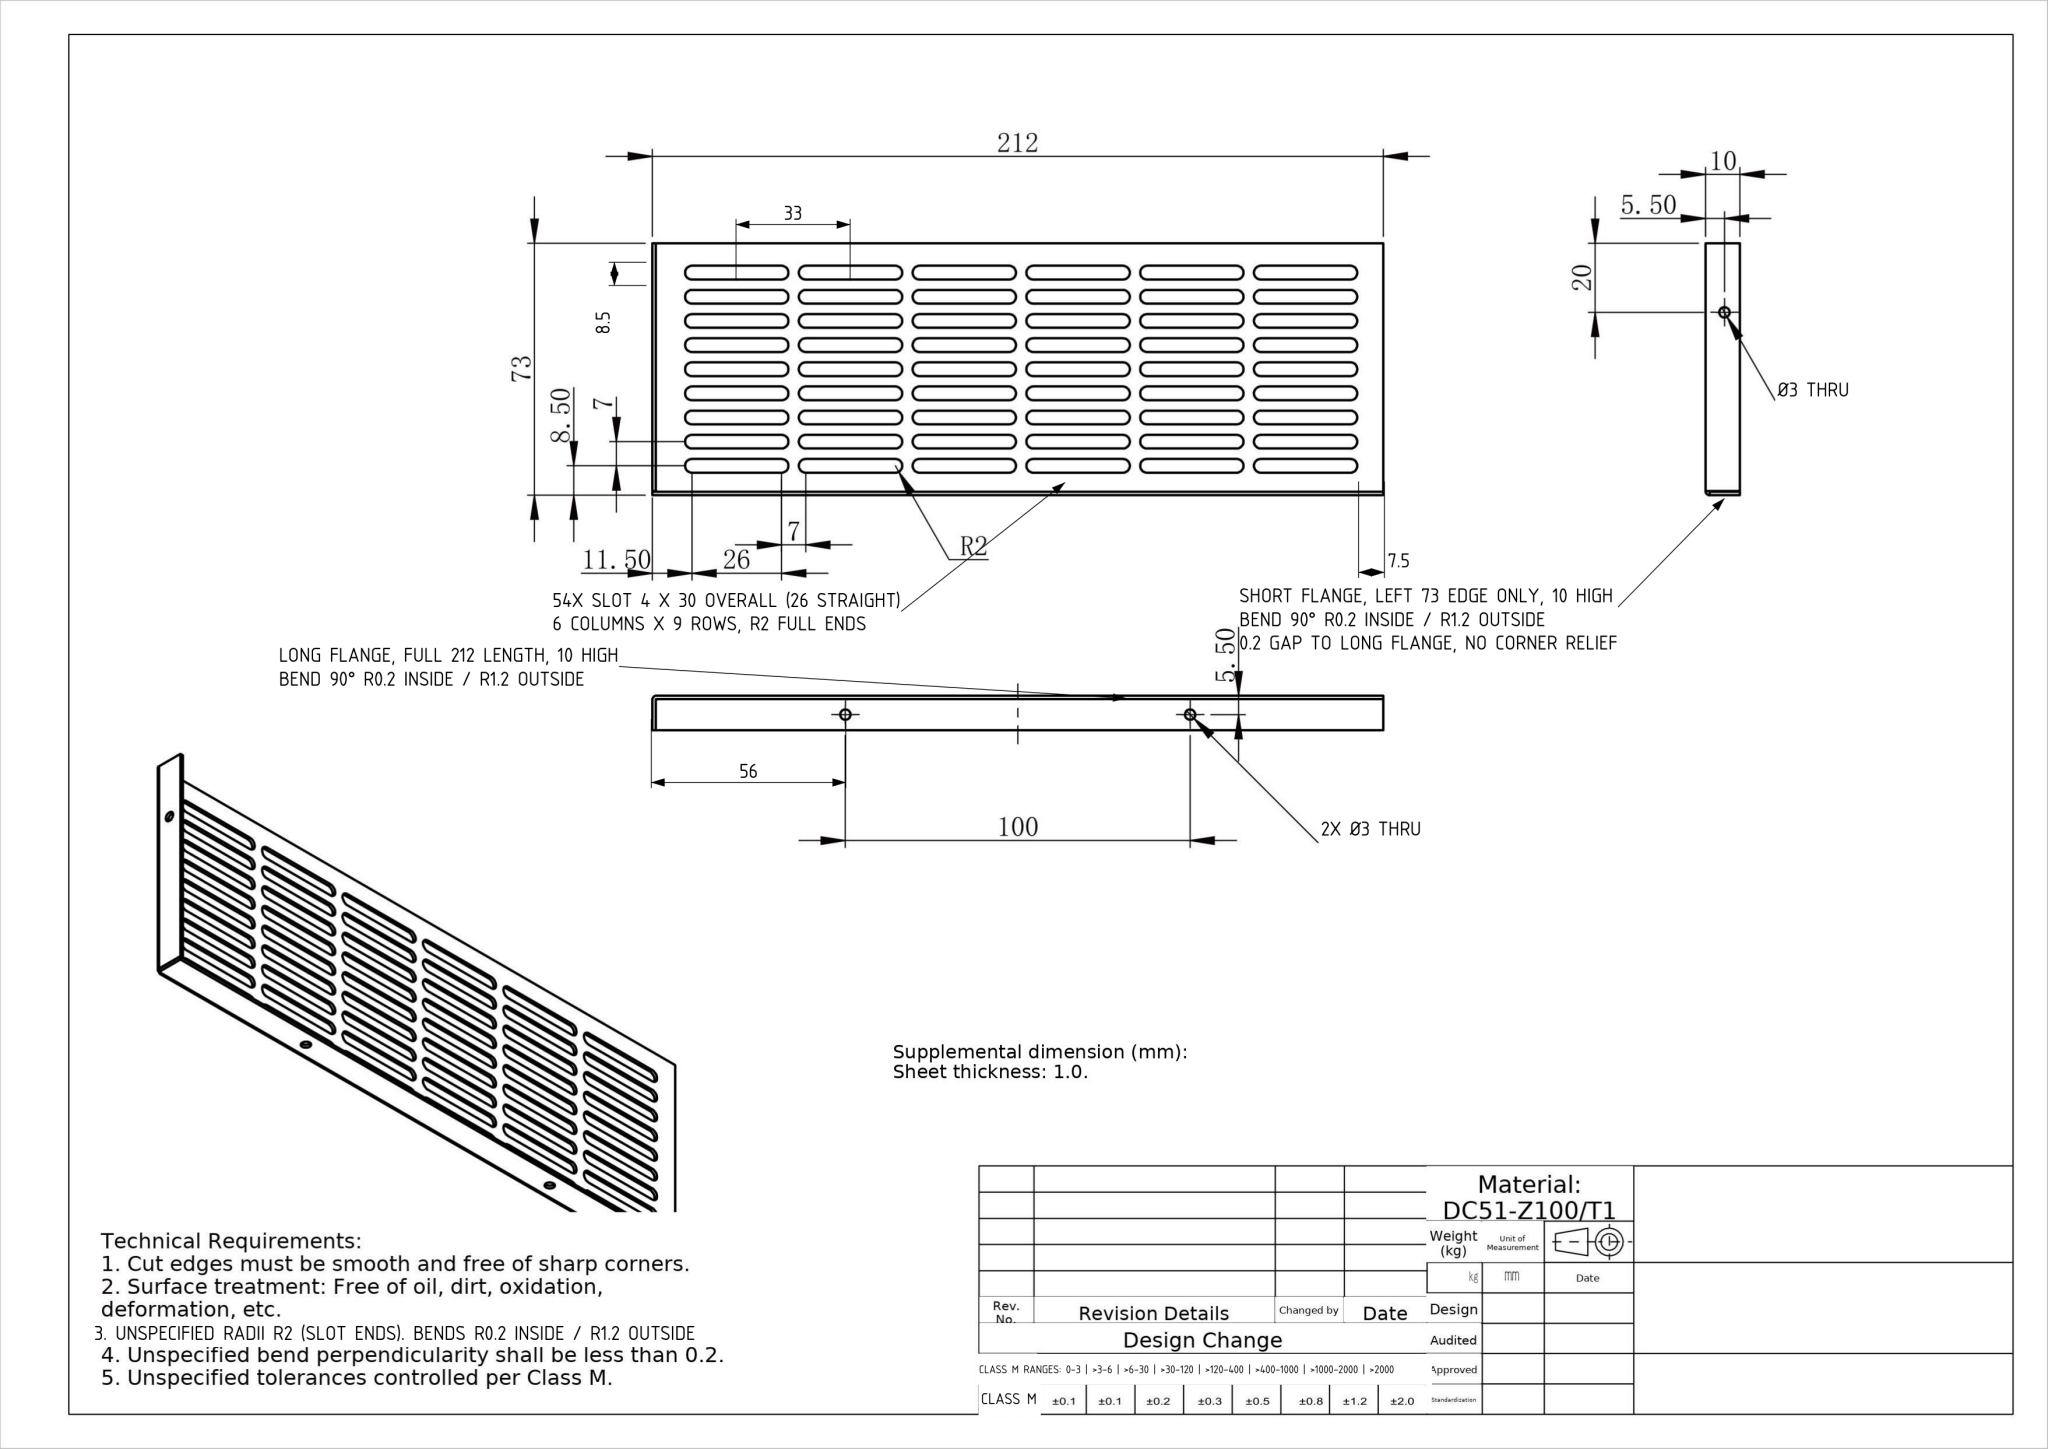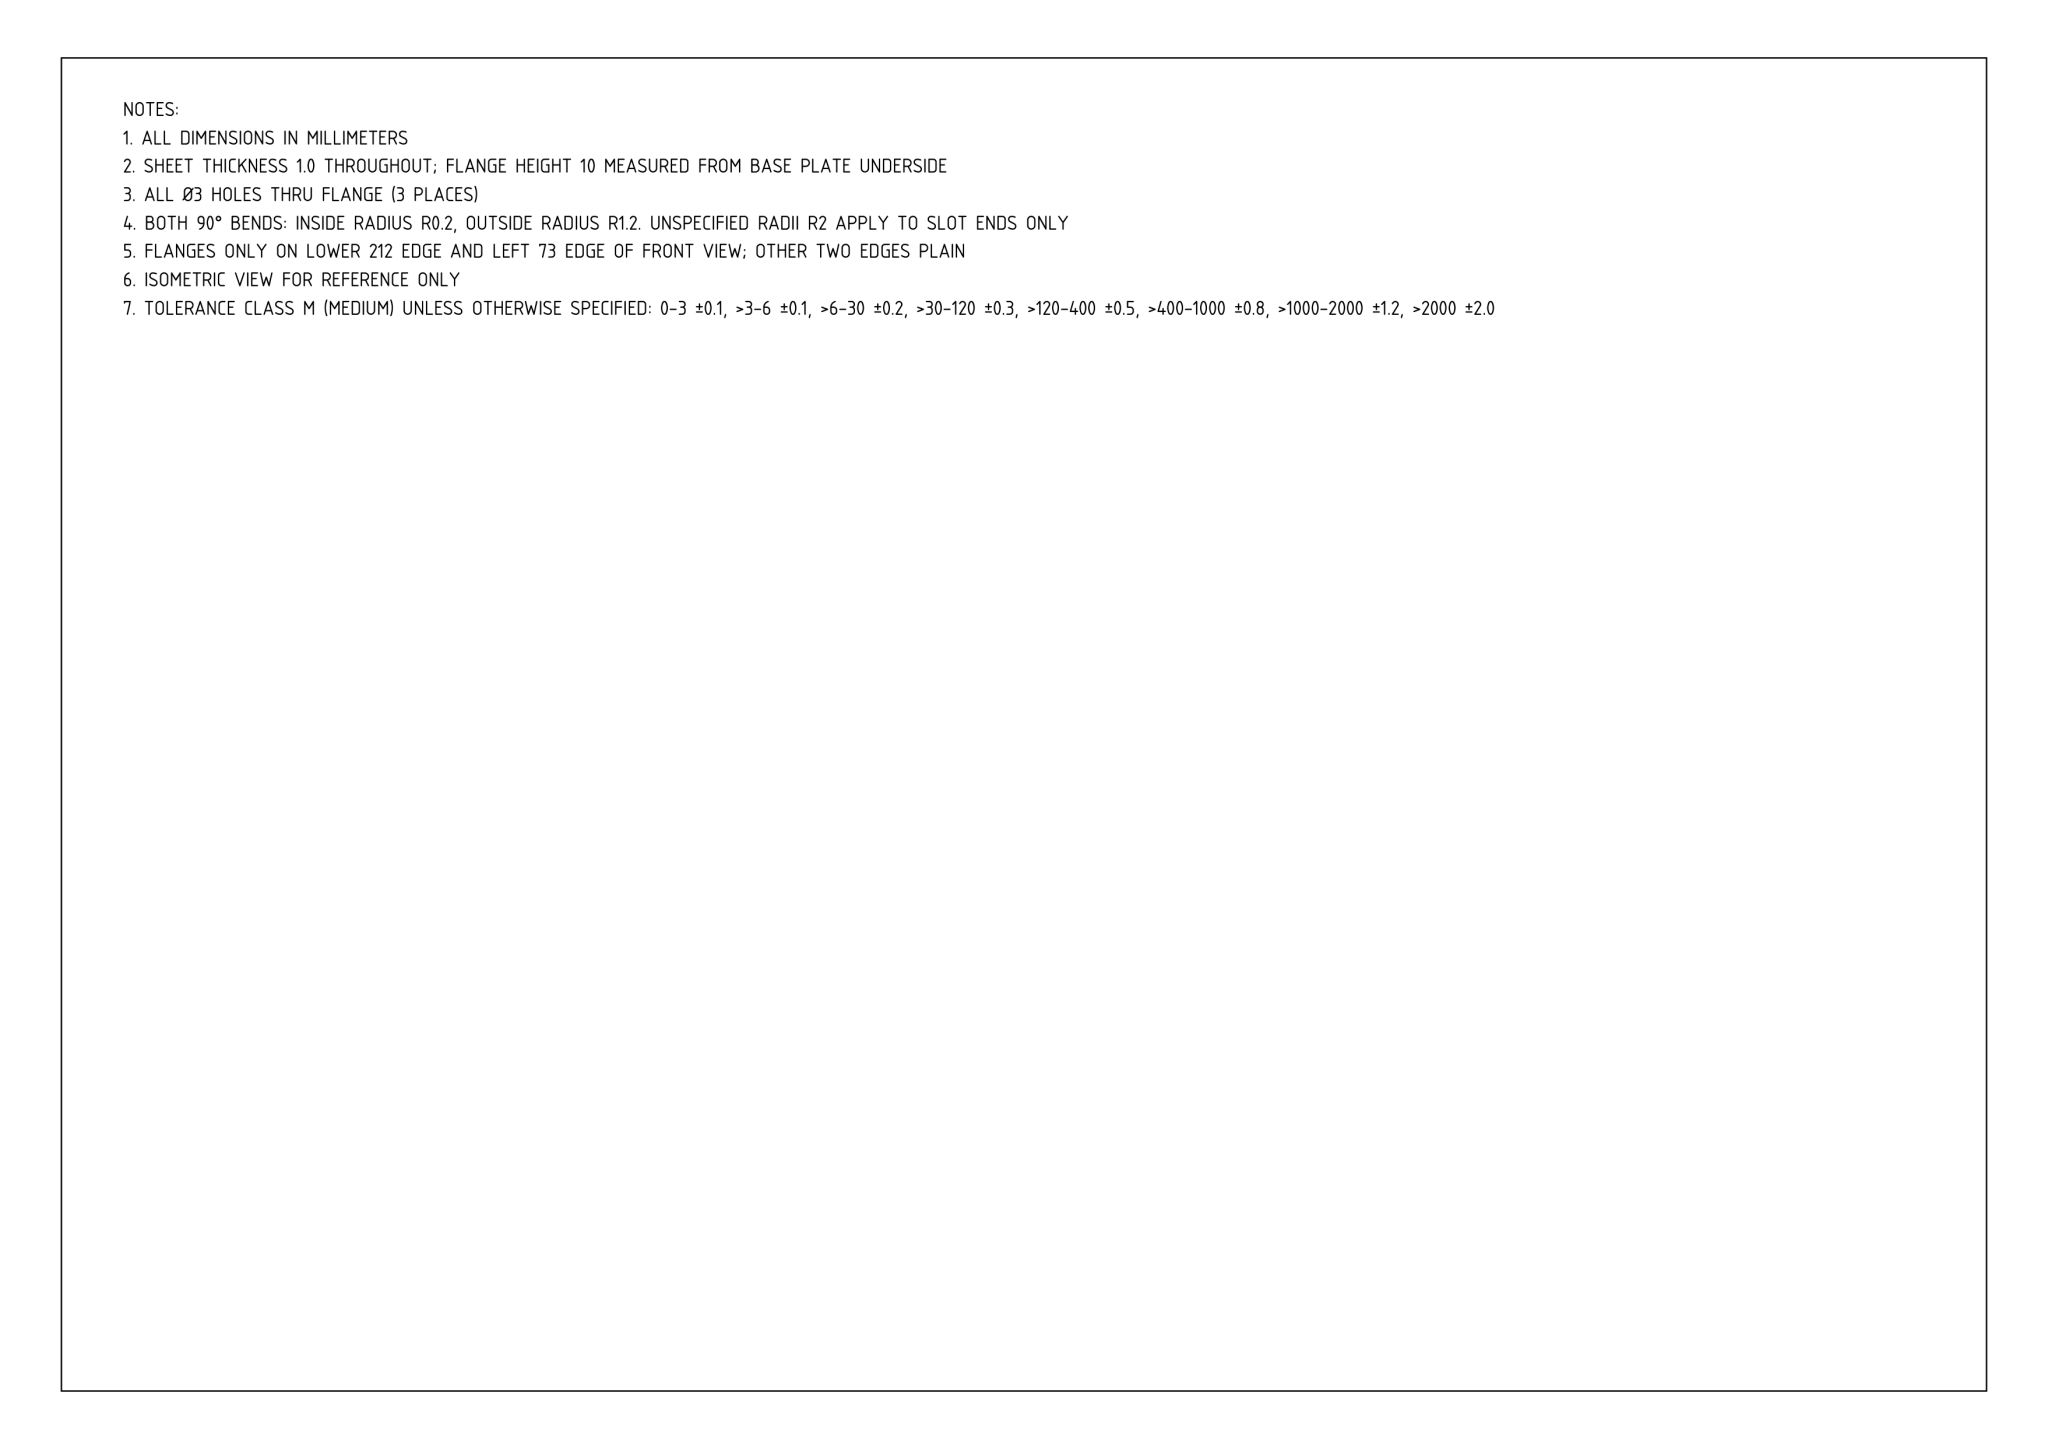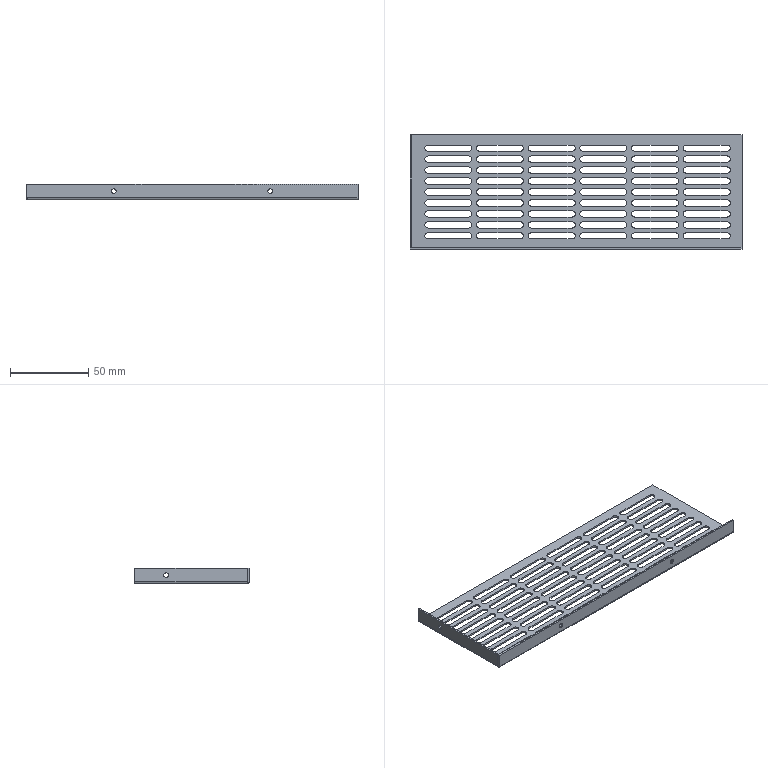Part | NX | mm | 1 solid | 299 faces | box 212 x 73 x 10 mm | volume 11628 mm3 | cylinder 172 | plane 127 | commonest cylinder face diameters 4 x162 3 x6 2.4 x2 0.4 x2